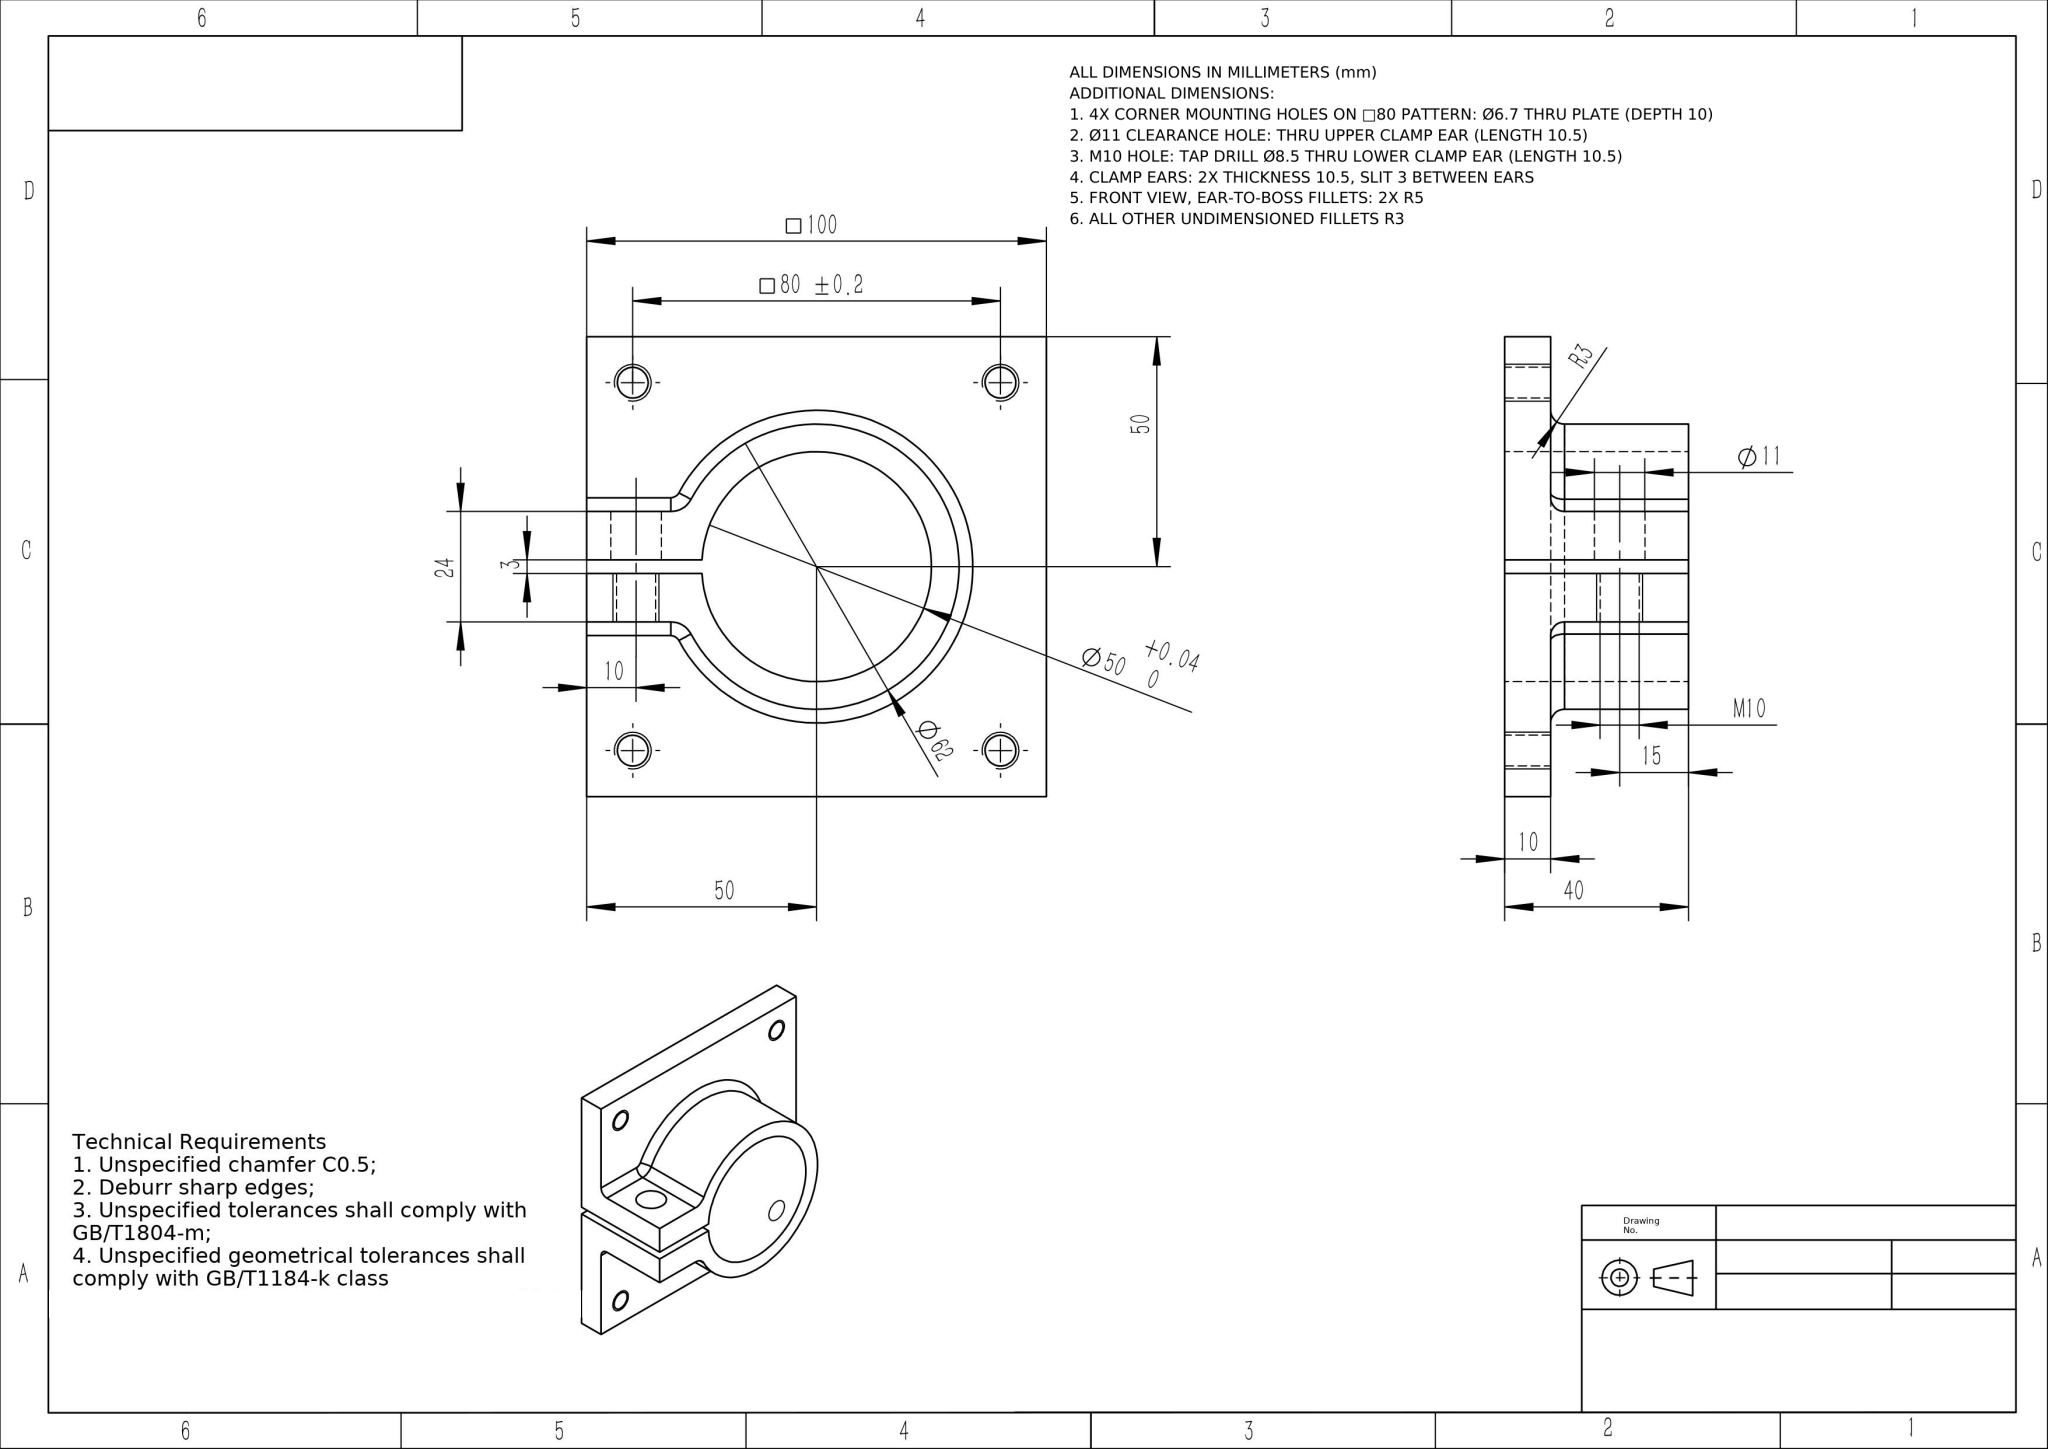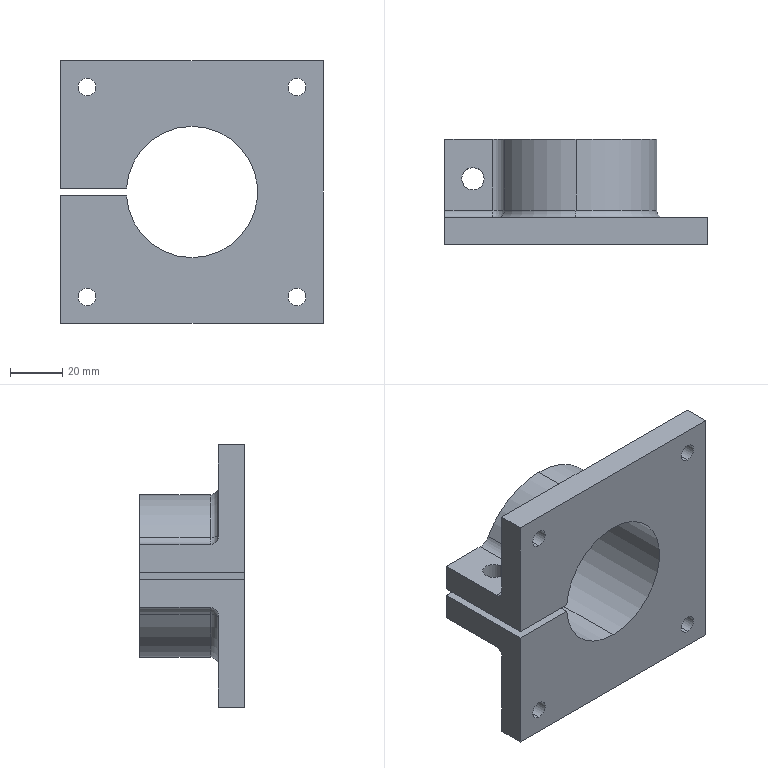Part | NX | mm | 1 solid | 39 faces | box 100 x 40 x 100 mm | volume 120787 mm3 | cylinder 22 | plane 12 | torus 5 | commonest cylinder face diameters 6.7 x8 50 x3 62 x3 11 x2 8.5 x2 10 x2 6 x2